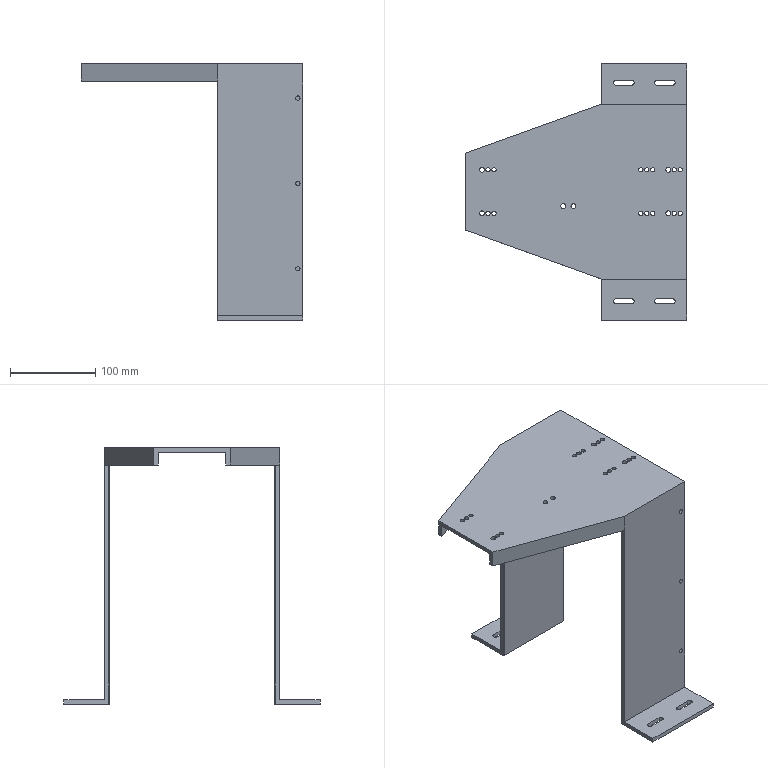Component | NX | SUPPORT_PLATE | 1 solid | 61 faces | volume 583397 mm3 | cylinder 31 | plane 30 | commonest cylinder face diameters 5 x17 6 x8 5.795 x6